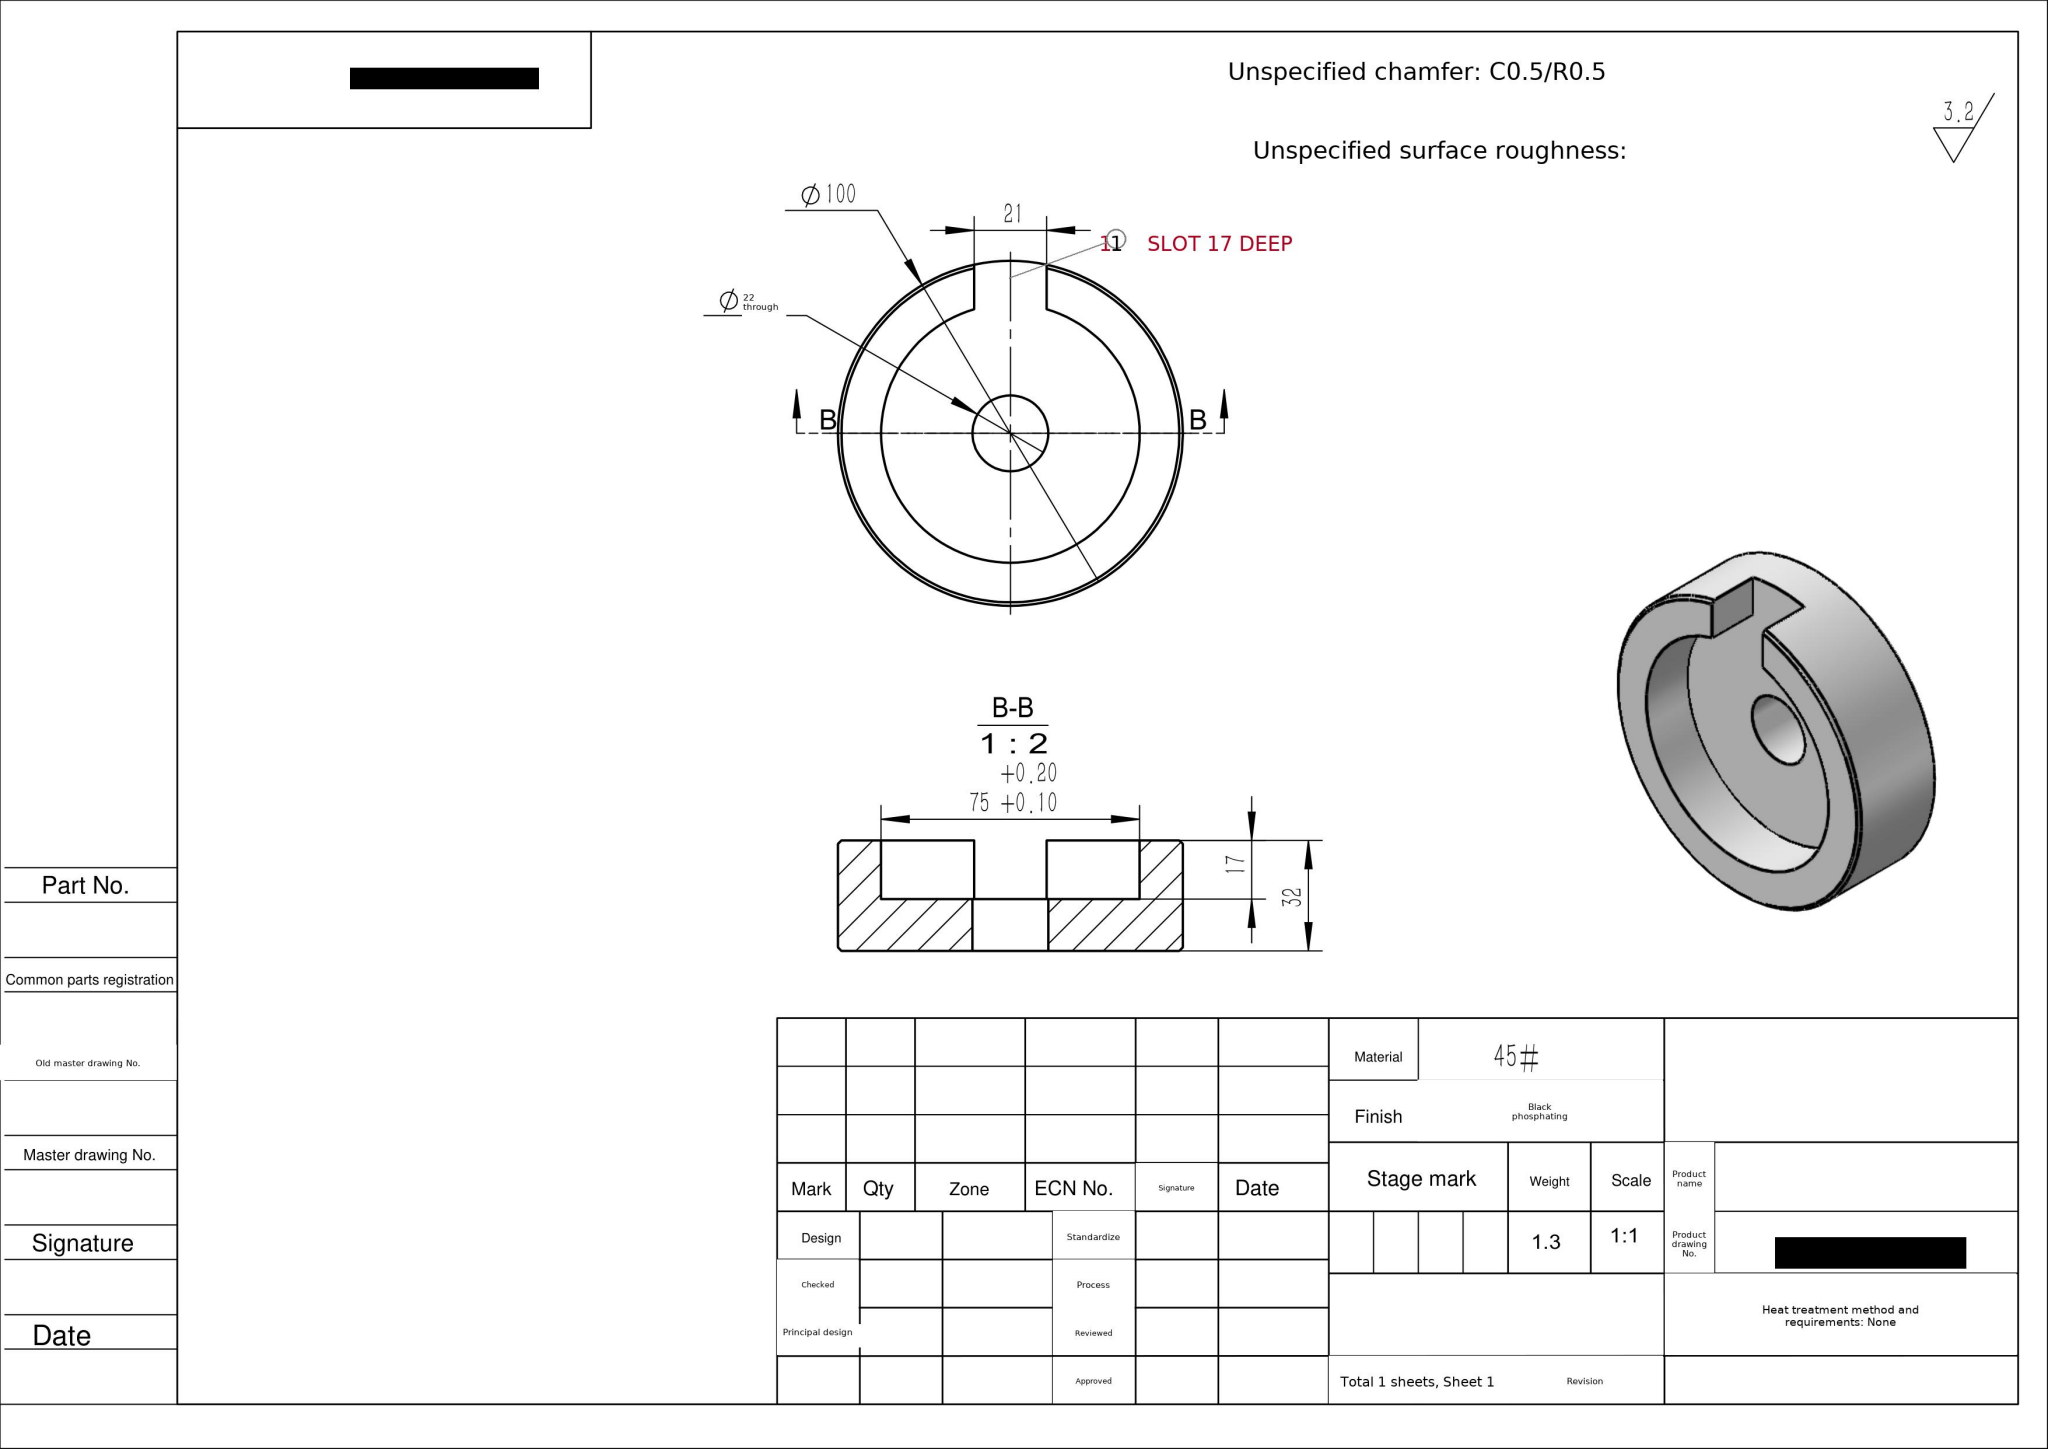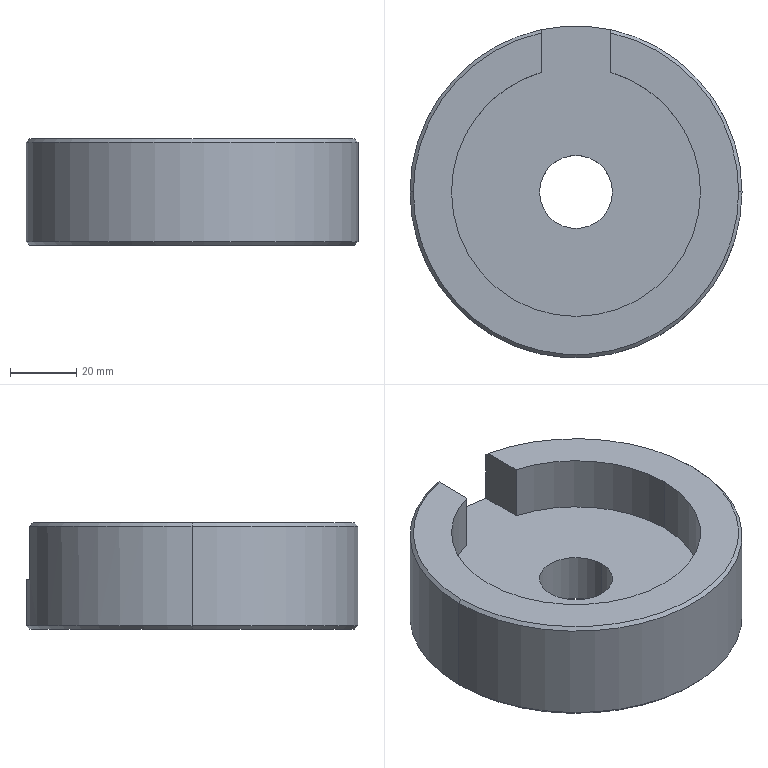Part | SolidWorks | mm | material 45# | 1 solid | 17 faces | box 100 x 100 x 32 mm | volume 165713 mm3 | cylinder 7 | cone 5 | plane 5 | commonest cylinder face diameters 75 x3 22 x2 100 x2
build123d program:
from build123d import *

# Parameters (mm, degrees)
SKETCH1_R             = 50
BOSS_EXTRUDE1_DEPTH   = 15
M20_CLEARANCE_HOLE1_D = 22
SKETCH4_R             = 50
SKETCH4_R_2           = 37.5
BOSS_EXTRUDE2_DEPTH   = 17
CHAMFER1_SIZE         = 1
SKETCH5_W             = 21
SKETCH5_H             = 65.178
CUT_EXTRUDE1_DEPTH    = 17


with BuildPart() as part:
    # Sketch1 → Boss-Extrude1 (new body)
    with BuildSketch(Plane.XY):
        Circle(SKETCH1_R)
    extrude(amount=BOSS_EXTRUDE1_DEPTH)

    # M20 Clearance Hole1 (through all)
    with Locations(Plane.XY.offset(15)):
        with Locations((0, 0)):
            Hole(M20_CLEARANCE_HOLE1_D / 2)

    # Sketch4 → Boss-Extrude2 (add)
    with BuildSketch(Plane.XY.offset(15)):
        Circle(SKETCH4_R)
        Circle(SKETCH4_R_2, mode=Mode.SUBTRACT)
    extrude(amount=BOSS_EXTRUDE2_DEPTH)

    # Chamfer1
    chamfer1_edges = [part.edges().sort_by_distance(p)[0] for p in [
        (-50, 0, 32),
        (-50, 0, 0),
    ]]
    chamfer(chamfer1_edges, length=CHAMFER1_SIZE)

    # Sketch5 → Cut-Extrude1 (cut)
    with BuildSketch(Plane.XY.offset(32)):
        with Locations((0, 32.589)):
            Rectangle(SKETCH5_W, SKETCH5_H)
    extrude(amount=-CUT_EXTRUDE1_DEPTH, mode=Mode.SUBTRACT)


solid = part.part
STEP:
#1=CARTESIAN_POINT('',(49.,0.,32.));
#2=VERTEX_POINT('',#1);
#3=CARTESIAN_POINT('',(10.5,47.862,32.));
#4=VERTEX_POINT('',#3);
#5=CARTESIAN_POINT('',(0.,0.,32.));
#6=DIRECTION('',(0.,0.,1.));
#7=DIRECTION('',(1.,0.,0.));
#8=AXIS2_PLACEMENT_3D('',#5,#6,#7);
#9=CIRCLE('',#8,49.);
#10=EDGE_CURVE('',#2,#4,#9,.T.);
#11=ORIENTED_EDGE('',*,*,#10,.F.);
#12=CARTESIAN_POINT('',(50.,0.,31.));
#13=VERTEX_POINT('',#12);
#14=CARTESIAN_POINT('',(49.,0.,32.));
#15=DIRECTION('',(0.7071,0.,-0.7071));
#16=VECTOR('',#15,1000.);
#17=LINE('',#14,#16);
#18=EDGE_CURVE('',#2,#13,#17,.T.);
#19=ORIENTED_EDGE('',*,*,#18,.T.);
#20=CARTESIAN_POINT('',(10.5,48.885,31.));
#21=VERTEX_POINT('',#20);
#22=CARTESIAN_POINT('',(0.,0.,31.));
#23=DIRECTION('',(0.,0.,-1.));
#24=DIRECTION('',(1.,0.,0.));
#25=AXIS2_PLACEMENT_3D('',#22,#23,#24);
#26=CIRCLE('',#25,50.);
#27=EDGE_CURVE('',#21,#13,#26,.T.);
#28=ORIENTED_EDGE('',*,*,#27,.F.);
#29=CARTESIAN_POINT('',(10.5,47.862,32.));
#30=CARTESIAN_POINT('',(10.5,48.203,31.667));
#31=CARTESIAN_POINT('',(10.5,48.544,31.333));
#32=CARTESIAN_POINT('',(10.5,48.885,31.));
#33=B_SPLINE_CURVE_WITH_KNOTS('',3,(#29,#30,#31,#32),.UNSPECIFIED.,.F.,.F.,(4,4),(0.04568,0.04711),.UNSPECIFIED.);
#34=EDGE_CURVE('',#4,#21,#33,.T.);
#35=ORIENTED_EDGE('',*,*,#34,.F.);
#36=EDGE_LOOP('',(#11,#19,#28,#35));
#37=FACE_OUTER_BOUND('',#36,.T.);
#38=CARTESIAN_POINT('',(0.,0.,32.));
#39=DIRECTION('',(0.,0.,-1.));
#40=DIRECTION('',(-1.,0.,0.));
#41=AXIS2_PLACEMENT_3D('',#38,#39,#40);
#42=CONICAL_SURFACE('',#41,49.,0.7854);
#43=ADVANCED_FACE('',(#37),#42,.T.);
#44=ORIENTED_EDGE('',*,*,#18,.F.);
#45=CARTESIAN_POINT('',(-49.,0.,32.));
#46=VERTEX_POINT('',#45);
#47=CARTESIAN_POINT('',(0.,0.,32.));
#48=DIRECTION('',(0.,0.,1.));
#49=DIRECTION('',(1.,0.,0.));
#50=AXIS2_PLACEMENT_3D('',#47,#48,#49);
#51=CIRCLE('',#50,49.);
#52=EDGE_CURVE('',#46,#2,#51,.T.);
#53=ORIENTED_EDGE('',*,*,#52,.F.);
#54=CARTESIAN_POINT('',(-50.,0.,31.));
#55=VERTEX_POINT('',#54);
#56=CARTESIAN_POINT('',(-49.,0.,32.));
#57=DIRECTION('',(-0.7071,0.,-0.7071));
#58=VECTOR('',#57,1000.);
#59=LINE('',#56,#58);
#60=EDGE_CURVE('',#46,#55,#59,.T.);
#61=ORIENTED_EDGE('',*,*,#60,.T.);
#62=CARTESIAN_POINT('',(0.,0.,31.));
#63=DIRECTION('',(0.,0.,-1.));
#64=DIRECTION('',(1.,0.,0.));
#65=AXIS2_PLACEMENT_3D('',#62,#63,#64);
#66=CIRCLE('',#65,50.);
#67=EDGE_CURVE('',#13,#55,#66,.T.);
#68=ORIENTED_EDGE('',*,*,#67,.F.);
#69=EDGE_LOOP('',(#44,#53,#61,#68));
#70=FACE_OUTER_BOUND('',#69,.T.);
#71=CARTESIAN_POINT('',(0.,0.,32.));
#72=DIRECTION('',(0.,0.,-1.));
#73=DIRECTION('',(-1.,0.,0.));
#74=AXIS2_PLACEMENT_3D('',#71,#72,#73);
#75=CONICAL_SURFACE('',#74,49.,0.7854);
#76=ADVANCED_FACE('',(#70),#75,.T.);
#77=CARTESIAN_POINT('',(-49.,0.,0.));
#78=VERTEX_POINT('',#77);
#79=CARTESIAN_POINT('',(49.,0.,0.));
#80=VERTEX_POINT('',#79);
#81=CARTESIAN_POINT('',(0.,0.,0.));
#82=DIRECTION('',(0.,0.,-1.));
#83=DIRECTION('',(1.,0.,0.));
#84=AXIS2_PLACEMENT_3D('',#81,#82,#83);
#85=CIRCLE('',#84,49.);
#86=EDGE_CURVE('',#78,#80,#85,.T.);
#87=ORIENTED_EDGE('',*,*,#86,.F.);
#88=CARTESIAN_POINT('',(-50.,0.,1.));
#89=VERTEX_POINT('',#88);
#90=CARTESIAN_POINT('',(-50.,0.,1.));
#91=DIRECTION('',(-0.7071,0.,0.7071));
#92=VECTOR('',#91,1000.);
#93=LINE('',#90,#92);
#94=EDGE_CURVE('',#78,#89,#93,.T.);
#95=ORIENTED_EDGE('',*,*,#94,.T.);
#96=CARTESIAN_POINT('',(50.,0.,1.));
#97=VERTEX_POINT('',#96);
#98=CARTESIAN_POINT('',(0.,0.,1.));
#99=DIRECTION('',(0.,0.,1.));
#100=DIRECTION('',(1.,0.,0.));
#101=AXIS2_PLACEMENT_3D('',#98,#99,#100);
#102=CIRCLE('',#101,50.);
#103=EDGE_CURVE('',#97,#89,#102,.T.);
#104=ORIENTED_EDGE('',*,*,#103,.F.);
#105=CARTESIAN_POINT('',(50.,0.,1.));
#106=DIRECTION('',(0.7071,0.,0.7071));
#107=VECTOR('',#106,1000.);
#108=LINE('',#105,#107);
#109=EDGE_CURVE('',#80,#97,#108,.T.);
#110=ORIENTED_EDGE('',*,*,#109,.F.);
#111=EDGE_LOOP('',(#87,#95,#104,#110));
#112=FACE_OUTER_BOUND('',#111,.T.);
#113=CARTESIAN_POINT('',(0.,0.,1.));
#114=DIRECTION('',(0.,0.,1.));
#115=DIRECTION('',(1.,0.,0.));
#116=AXIS2_PLACEMENT_3D('',#113,#114,#115);
#117=CONICAL_SURFACE('',#116,50.,0.7854);
#118=ADVANCED_FACE('',(#112),#117,.T.);
#119=CARTESIAN_POINT('',(-37.5,0.,32.));
#120=VERTEX_POINT('',#119);
#121=CARTESIAN_POINT('',(37.5,0.,32.));
#122=VERTEX_POINT('',#121);
#123=CARTESIAN_POINT('',(0.,0.,32.));
#124=DIRECTION('',(0.,0.,1.));
#125=DIRECTION('',(1.,0.,0.));
#126=AXIS2_PLACEMENT_3D('',#123,#124,#125);
#127=CIRCLE('',#126,37.5);
#128=EDGE_CURVE('',#120,#122,#127,.T.);
#129=ORIENTED_EDGE('',*,*,#128,.T.);
#130=CARTESIAN_POINT('',(37.5,0.,15.));
#131=VERTEX_POINT('',#130);
#132=CARTESIAN_POINT('',(37.5,0.,32.));
#133=DIRECTION('',(0.,0.,-1.));
#134=VECTOR('',#133,1000.);
#135=LINE('',#132,#134);
#136=EDGE_CURVE('',#122,#131,#135,.T.);
#137=ORIENTED_EDGE('',*,*,#136,.T.);
#138=CARTESIAN_POINT('',(-37.5,0.,15.));
#139=VERTEX_POINT('',#138);
#140=CARTESIAN_POINT('',(0.,0.,15.));
#141=DIRECTION('',(0.,0.,-1.));
#142=DIRECTION('',(1.,0.,0.));
#143=AXIS2_PLACEMENT_3D('',#140,#141,#142);
#144=CIRCLE('',#143,37.5);
#145=EDGE_CURVE('',#131,#139,#144,.T.);
#146=ORIENTED_EDGE('',*,*,#145,.T.);
#147=CARTESIAN_POINT('',(-37.5,0.,32.));
#148=DIRECTION('',(0.,0.,-1.));
#149=VECTOR('',#148,1000.);
#150=LINE('',#147,#149);
#151=EDGE_CURVE('',#120,#139,#150,.T.);
#152=ORIENTED_EDGE('',*,*,#151,.F.);
#153=EDGE_LOOP('',(#129,#137,#146,#152));
#154=FACE_OUTER_BOUND('',#153,.T.);
#155=CARTESIAN_POINT('',(0.,0.,32.));
#156=DIRECTION('',(0.,0.,-1.));
#157=DIRECTION('',(-1.,0.,0.));
#158=AXIS2_PLACEMENT_3D('',#155,#156,#157);
#159=CYLINDRICAL_SURFACE('',#158,37.5);
#160=ADVANCED_FACE('',(#154),#159,.F.);
#161=CARTESIAN_POINT('',(-10.5,36.,32.));
#162=VERTEX_POINT('',#161);
#163=CARTESIAN_POINT('',(0.,0.,32.));
#164=DIRECTION('',(0.,0.,1.));
#165=DIRECTION('',(1.,0.,0.));
#166=AXIS2_PLACEMENT_3D('',#163,#164,#165);
#167=CIRCLE('',#166,37.5);
#168=EDGE_CURVE('',#162,#120,#167,.T.);
#169=ORIENTED_EDGE('',*,*,#168,.T.);
#170=ORIENTED_EDGE('',*,*,#151,.T.);
#171=CARTESIAN_POINT('',(-10.5,36.,15.));
#172=VERTEX_POINT('',#171);
#173=CARTESIAN_POINT('',(0.,0.,15.));
#174=DIRECTION('',(0.,0.,-1.));
#175=DIRECTION('',(1.,0.,0.));
#176=AXIS2_PLACEMENT_3D('',#173,#174,#175);
#177=CIRCLE('',#176,37.5);
#178=EDGE_CURVE('',#139,#172,#177,.T.);
#179=ORIENTED_EDGE('',*,*,#178,.T.);
#180=CARTESIAN_POINT('',(-10.5,36.,32.));
#181=DIRECTION('',(0.,0.,-1.));
#182=VECTOR('',#181,1000.);
#183=LINE('',#180,#182);
#184=EDGE_CURVE('',#162,#172,#183,.T.);
#185=ORIENTED_EDGE('',*,*,#184,.F.);
#186=EDGE_LOOP('',(#169,#170,#179,#185));
#187=FACE_OUTER_BOUND('',#186,.T.);
#188=CARTESIAN_POINT('',(0.,0.,32.));
#189=DIRECTION('',(0.,0.,-1.));
#190=DIRECTION('',(-1.,0.,0.));
#191=AXIS2_PLACEMENT_3D('',#188,#189,#190);
#192=CYLINDRICAL_SURFACE('',#191,37.5);
#193=ADVANCED_FACE('',(#187),#192,.F.);
#194=CARTESIAN_POINT('',(-11.,0.,0.));
#195=VERTEX_POINT('',#194);
#196=CARTESIAN_POINT('',(11.,0.,0.));
#197=VERTEX_POINT('',#196);
#198=CARTESIAN_POINT('',(0.,0.,0.));
#199=DIRECTION('',(0.,0.,1.));
#200=DIRECTION('',(1.,0.,0.));
#201=AXIS2_PLACEMENT_3D('',#198,#199,#200);
#202=CIRCLE('',#201,11.);
#203=EDGE_CURVE('',#195,#197,#202,.T.);
#204=ORIENTED_EDGE('',*,*,#203,.F.);
#205=CARTESIAN_POINT('',(-11.,0.,15.));
#206=VERTEX_POINT('',#205);
#207=CARTESIAN_POINT('',(-11.,0.,15.));
#208=DIRECTION('',(0.,0.,1.));
#209=VECTOR('',#208,1000.);
#210=LINE('',#207,#209);
#211=EDGE_CURVE('',#195,#206,#210,.T.);
#212=ORIENTED_EDGE('',*,*,#211,.T.);
#213=CARTESIAN_POINT('',(11.,0.,15.));
#214=VERTEX_POINT('',#213);
#215=CARTESIAN_POINT('',(0.,0.,15.));
#216=DIRECTION('',(0.,0.,1.));
#217=DIRECTION('',(1.,0.,0.));
#218=AXIS2_PLACEMENT_3D('',#215,#216,#217);
#219=CIRCLE('',#218,11.);
#220=EDGE_CURVE('',#206,#214,#219,.T.);
#221=ORIENTED_EDGE('',*,*,#220,.T.);
#222=CARTESIAN_POINT('',(11.,0.,15.));
#223=DIRECTION('',(0.,0.,1.));
#224=VECTOR('',#223,1000.);
#225=LINE('',#222,#224);
#226=EDGE_CURVE('',#197,#214,#225,.T.);
#227=ORIENTED_EDGE('',*,*,#226,.F.);
#228=EDGE_LOOP('',(#204,#212,#221,#227));
#229=FACE_OUTER_BOUND('',#228,.T.);
#230=CARTESIAN_POINT('',(0.,0.,15.));
#231=DIRECTION('',(0.,0.,1.));
#232=DIRECTION('',(1.,0.,0.));
#233=AXIS2_PLACEMENT_3D('',#230,#231,#232);
#234=CYLINDRICAL_SURFACE('',#233,11.);
#235=ADVANCED_FACE('',(#229),#234,.F.);
#236=ORIENTED_EDGE('',*,*,#27,.T.);
#237=CARTESIAN_POINT('',(50.,0.,15.));
#238=DIRECTION('',(0.,0.,-1.));
#239=VECTOR('',#238,1000.);
#240=LINE('',#237,#239);
#241=EDGE_CURVE('',#13,#97,#240,.T.);
#242=ORIENTED_EDGE('',*,*,#241,.T.);
#243=ORIENTED_EDGE('',*,*,#103,.T.);
#244=CARTESIAN_POINT('',(-50.,0.,15.));
#245=DIRECTION('',(0.,0.,-1.));
#246=VECTOR('',#245,1000.);
#247=LINE('',#244,#246);
#248=EDGE_CURVE('',#55,#89,#247,.T.);
#249=ORIENTED_EDGE('',*,*,#248,.F.);
#250=CARTESIAN_POINT('',(-10.5,48.885,31.));
#251=VERTEX_POINT('',#250);
#252=CARTESIAN_POINT('',(0.,0.,31.));
#253=DIRECTION('',(0.,0.,-1.));
#254=DIRECTION('',(1.,0.,0.));
#255=AXIS2_PLACEMENT_3D('',#252,#253,#254);
#256=CIRCLE('',#255,50.);
#257=EDGE_CURVE('',#55,#251,#256,.T.);
#258=ORIENTED_EDGE('',*,*,#257,.T.);
#259=CARTESIAN_POINT('',(-10.5,48.885,15.));
#260=VERTEX_POINT('',#259);
#261=CARTESIAN_POINT('',(-10.5,48.885,15.));
#262=DIRECTION('',(0.,0.,-1.));
#263=VECTOR('',#262,1000.);
#264=LINE('',#261,#263);
#265=EDGE_CURVE('',#251,#260,#264,.T.);
#266=ORIENTED_EDGE('',*,*,#265,.T.);
#267=CARTESIAN_POINT('',(10.5,48.885,15.));
#268=VERTEX_POINT('',#267);
#269=CARTESIAN_POINT('',(0.,0.,15.));
#270=DIRECTION('',(0.,0.,1.));
#271=DIRECTION('',(1.,0.,0.));
#272=AXIS2_PLACEMENT_3D('',#269,#270,#271);
#273=CIRCLE('',#272,50.);
#274=EDGE_CURVE('',#268,#260,#273,.T.);
#275=ORIENTED_EDGE('',*,*,#274,.F.);
#276=CARTESIAN_POINT('',(10.5,48.885,15.));
#277=DIRECTION('',(0.,0.,1.));
#278=VECTOR('',#277,1000.);
#279=LINE('',#276,#278);
#280=EDGE_CURVE('',#268,#21,#279,.T.);
#281=ORIENTED_EDGE('',*,*,#280,.T.);
#282=EDGE_LOOP('',(#236,#242,#243,#249,#258,#266,#275,#281));
#283=FACE_OUTER_BOUND('',#282,.T.);
#284=CARTESIAN_POINT('',(0.,0.,15.));
#285=DIRECTION('',(0.,0.,-1.));
#286=DIRECTION('',(-1.,0.,0.));
#287=AXIS2_PLACEMENT_3D('',#284,#285,#286);
#288=CYLINDRICAL_SURFACE('',#287,50.);
#289=ADVANCED_FACE('',(#283),#288,.T.);
#290=CARTESIAN_POINT('',(10.5,36.,15.));
#291=VERTEX_POINT('',#290);
#292=CARTESIAN_POINT('',(0.,0.,15.));
#293=DIRECTION('',(0.,0.,-1.));
#294=DIRECTION('',(1.,0.,0.));
#295=AXIS2_PLACEMENT_3D('',#292,#293,#294);
#296=CIRCLE('',#295,37.5);
#297=EDGE_CURVE('',#291,#131,#296,.T.);
#298=ORIENTED_EDGE('',*,*,#297,.F.);
#299=CARTESIAN_POINT('',(10.5,-0.,15.));
#300=DIRECTION('',(-0.,-1.,0.));
#301=VECTOR('',#300,1000.);
#302=LINE('',#299,#301);
#303=EDGE_CURVE('',#268,#291,#302,.T.);
#304=ORIENTED_EDGE('',*,*,#303,.F.);
#305=ORIENTED_EDGE('',*,*,#274,.T.);
#306=CARTESIAN_POINT('',(-10.5,-0.,15.));
#307=DIRECTION('',(-0.,1.,0.));
#308=VECTOR('',#307,1000.);
#309=LINE('',#306,#308);
#310=EDGE_CURVE('',#172,#260,#309,.T.);
#311=ORIENTED_EDGE('',*,*,#310,.F.);
#312=ORIENTED_EDGE('',*,*,#178,.F.);
#313=ORIENTED_EDGE('',*,*,#145,.F.);
#314=EDGE_LOOP('',(#298,#304,#305,#311,#312,#313));
#315=FACE_OUTER_BOUND('',#314,.T.);
#316=CARTESIAN_POINT('',(0.,0.,15.));
#317=DIRECTION('',(0.,0.,1.));
#318=DIRECTION('',(1.,0.,0.));
#319=AXIS2_PLACEMENT_3D('',#316,#317,#318);
#320=CIRCLE('',#319,11.);
#321=EDGE_CURVE('',#214,#206,#320,.T.);
#322=ORIENTED_EDGE('',*,*,#321,.F.);
#323=ORIENTED_EDGE('',*,*,#220,.F.);
#324=EDGE_LOOP('',(#322,#323));
#325=FACE_BOUND('',#324,.T.);
#326=CARTESIAN_POINT('',(0.,0.,15.));
#327=DIRECTION('',(0.,0.,1.));
#328=DIRECTION('',(1.,0.,0.));
#329=AXIS2_PLACEMENT_3D('',#326,#327,#328);
#330=PLANE('',#329);
#331=ADVANCED_FACE('',(#315,#325),#330,.T.);
#332=ORIENTED_EDGE('',*,*,#241,.F.);
#333=ORIENTED_EDGE('',*,*,#67,.T.);
#334=ORIENTED_EDGE('',*,*,#248,.T.);
#335=CARTESIAN_POINT('',(0.,0.,1.));
#336=DIRECTION('',(0.,0.,1.));
#337=DIRECTION('',(1.,0.,0.));
#338=AXIS2_PLACEMENT_3D('',#335,#336,#337);
#339=CIRCLE('',#338,50.);
#340=EDGE_CURVE('',#89,#97,#339,.T.);
#341=ORIENTED_EDGE('',*,*,#340,.T.);
#342=EDGE_LOOP('',(#332,#333,#334,#341));
#343=FACE_OUTER_BOUND('',#342,.T.);
#344=CARTESIAN_POINT('',(0.,0.,15.));
#345=DIRECTION('',(0.,0.,-1.));
#346=DIRECTION('',(-1.,0.,0.));
#347=AXIS2_PLACEMENT_3D('',#344,#345,#346);
#348=CYLINDRICAL_SURFACE('',#347,50.);
#349=ADVANCED_FACE('',(#343),#348,.T.);
#350=CARTESIAN_POINT('',(0.,0.,0.));
#351=DIRECTION('',(0.,0.,-1.));
#352=DIRECTION('',(1.,0.,0.));
#353=AXIS2_PLACEMENT_3D('',#350,#351,#352);
#354=CIRCLE('',#353,49.);
#355=EDGE_CURVE('',#80,#78,#354,.T.);
#356=ORIENTED_EDGE('',*,*,#355,.T.);
#357=ORIENTED_EDGE('',*,*,#86,.T.);
#358=EDGE_LOOP('',(#356,#357));
#359=FACE_OUTER_BOUND('',#358,.T.);
#360=CARTESIAN_POINT('',(0.,0.,0.));
#361=DIRECTION('',(0.,0.,1.));
#362=DIRECTION('',(1.,0.,0.));
#363=AXIS2_PLACEMENT_3D('',#360,#361,#362);
#364=CIRCLE('',#363,11.);
#365=EDGE_CURVE('',#197,#195,#364,.T.);
#366=ORIENTED_EDGE('',*,*,#365,.T.);
#367=ORIENTED_EDGE('',*,*,#203,.T.);
#368=EDGE_LOOP('',(#366,#367));
#369=FACE_BOUND('',#368,.T.);
#370=CARTESIAN_POINT('',(0.,0.,0.));
#371=DIRECTION('',(0.,0.,1.));
#372=DIRECTION('',(1.,0.,0.));
#373=AXIS2_PLACEMENT_3D('',#370,#371,#372);
#374=PLANE('',#373);
#375=ADVANCED_FACE('',(#359,#369),#374,.F.);
#376=ORIENTED_EDGE('',*,*,#211,.F.);
#377=ORIENTED_EDGE('',*,*,#365,.F.);
#378=ORIENTED_EDGE('',*,*,#226,.T.);
#379=ORIENTED_EDGE('',*,*,#321,.T.);
#380=EDGE_LOOP('',(#376,#377,#378,#379));
#381=FACE_OUTER_BOUND('',#380,.T.);
#382=CARTESIAN_POINT('',(0.,0.,15.));
#383=DIRECTION('',(0.,0.,1.));
#384=DIRECTION('',(1.,0.,0.));
#385=AXIS2_PLACEMENT_3D('',#382,#383,#384);
#386=CYLINDRICAL_SURFACE('',#385,11.);
#387=ADVANCED_FACE('',(#381),#386,.F.);
#388=CARTESIAN_POINT('',(10.5,36.,32.));
#389=VERTEX_POINT('',#388);
#390=CARTESIAN_POINT('',(10.5,-0.,32.));
#391=DIRECTION('',(0.,1.,0.));
#392=VECTOR('',#391,1000.);
#393=LINE('',#390,#392);
#394=EDGE_CURVE('',#389,#4,#393,.T.);
#395=ORIENTED_EDGE('',*,*,#394,.F.);
#396=CARTESIAN_POINT('',(0.,0.,32.));
#397=DIRECTION('',(0.,0.,1.));
#398=DIRECTION('',(1.,0.,0.));
#399=AXIS2_PLACEMENT_3D('',#396,#397,#398);
#400=CIRCLE('',#399,37.5);
#401=EDGE_CURVE('',#122,#389,#400,.T.);
#402=ORIENTED_EDGE('',*,*,#401,.F.);
#403=ORIENTED_EDGE('',*,*,#128,.F.);
#404=ORIENTED_EDGE('',*,*,#168,.F.);
#405=CARTESIAN_POINT('',(-10.5,47.862,32.));
#406=VERTEX_POINT('',#405);
#407=CARTESIAN_POINT('',(-10.5,-0.,32.));
#408=DIRECTION('',(0.,-1.,0.));
#409=VECTOR('',#408,1000.);
#410=LINE('',#407,#409);
#411=EDGE_CURVE('',#406,#162,#410,.T.);
#412=ORIENTED_EDGE('',*,*,#411,.F.);
#413=CARTESIAN_POINT('',(0.,0.,32.));
#414=DIRECTION('',(0.,0.,1.));
#415=DIRECTION('',(1.,0.,0.));
#416=AXIS2_PLACEMENT_3D('',#413,#414,#415);
#417=CIRCLE('',#416,49.);
#418=EDGE_CURVE('',#406,#46,#417,.T.);
#419=ORIENTED_EDGE('',*,*,#418,.T.);
#420=ORIENTED_EDGE('',*,*,#52,.T.);
#421=ORIENTED_EDGE('',*,*,#10,.T.);
#422=EDGE_LOOP('',(#395,#402,#403,#404,#412,#419,#420,#421));
#423=FACE_OUTER_BOUND('',#422,.T.);
#424=CARTESIAN_POINT('',(0.,0.,32.));
#425=DIRECTION('',(0.,0.,1.));
#426=DIRECTION('',(1.,0.,0.));
#427=AXIS2_PLACEMENT_3D('',#424,#425,#426);
#428=PLANE('',#427);
#429=ADVANCED_FACE('',(#423),#428,.T.);
#430=ORIENTED_EDGE('',*,*,#136,.F.);
#431=ORIENTED_EDGE('',*,*,#401,.T.);
#432=CARTESIAN_POINT('',(10.5,36.,32.));
#433=DIRECTION('',(0.,0.,1.));
#434=VECTOR('',#433,1000.);
#435=LINE('',#432,#434);
#436=EDGE_CURVE('',#291,#389,#435,.T.);
#437=ORIENTED_EDGE('',*,*,#436,.F.);
#438=ORIENTED_EDGE('',*,*,#297,.T.);
#439=EDGE_LOOP('',(#430,#431,#437,#438));
#440=FACE_OUTER_BOUND('',#439,.T.);
#441=CARTESIAN_POINT('',(0.,0.,32.));
#442=DIRECTION('',(0.,0.,-1.));
#443=DIRECTION('',(-1.,0.,0.));
#444=AXIS2_PLACEMENT_3D('',#441,#442,#443);
#445=CYLINDRICAL_SURFACE('',#444,37.5);
#446=ADVANCED_FACE('',(#440),#445,.F.);
#447=ORIENTED_EDGE('',*,*,#94,.F.);
#448=ORIENTED_EDGE('',*,*,#355,.F.);
#449=ORIENTED_EDGE('',*,*,#109,.T.);
#450=ORIENTED_EDGE('',*,*,#340,.F.);
#451=EDGE_LOOP('',(#447,#448,#449,#450));
#452=FACE_OUTER_BOUND('',#451,.T.);
#453=CARTESIAN_POINT('',(0.,0.,1.));
#454=DIRECTION('',(0.,0.,1.));
#455=DIRECTION('',(1.,0.,0.));
#456=AXIS2_PLACEMENT_3D('',#453,#454,#455);
#457=CONICAL_SURFACE('',#456,50.,0.7854);
#458=ADVANCED_FACE('',(#452),#457,.T.);
#459=ORIENTED_EDGE('',*,*,#60,.F.);
#460=ORIENTED_EDGE('',*,*,#418,.F.);
#461=CARTESIAN_POINT('',(-10.5,48.885,31.));
#462=CARTESIAN_POINT('',(-10.5,48.544,31.333));
#463=CARTESIAN_POINT('',(-10.5,48.203,31.667));
#464=CARTESIAN_POINT('',(-10.5,47.862,32.));
#465=B_SPLINE_CURVE_WITH_KNOTS('',3,(#461,#462,#463,#464),.UNSPECIFIED.,.F.,.F.,(4,4),(0.05125,0.05268),.UNSPECIFIED.);
#466=EDGE_CURVE('',#251,#406,#465,.T.);
#467=ORIENTED_EDGE('',*,*,#466,.F.);
#468=ORIENTED_EDGE('',*,*,#257,.F.);
#469=EDGE_LOOP('',(#459,#460,#467,#468));
#470=FACE_OUTER_BOUND('',#469,.T.);
#471=CARTESIAN_POINT('',(0.,0.,32.));
#472=DIRECTION('',(0.,0.,-1.));
#473=DIRECTION('',(-1.,0.,0.));
#474=AXIS2_PLACEMENT_3D('',#471,#472,#473);
#475=CONICAL_SURFACE('',#474,49.,0.7854);
#476=ADVANCED_FACE('',(#470),#475,.T.);
#477=ORIENTED_EDGE('',*,*,#436,.T.);
#478=ORIENTED_EDGE('',*,*,#394,.T.);
#479=ORIENTED_EDGE('',*,*,#34,.T.);
#480=ORIENTED_EDGE('',*,*,#280,.F.);
#481=ORIENTED_EDGE('',*,*,#303,.T.);
#482=EDGE_LOOP('',(#477,#478,#479,#480,#481));
#483=FACE_OUTER_BOUND('',#482,.T.);
#484=CARTESIAN_POINT('',(10.5,-0.,-53.478));
#485=DIRECTION('',(1.,-0.,0.));
#486=DIRECTION('',(0.,1.,0.));
#487=AXIS2_PLACEMENT_3D('',#484,#485,#486);
#488=PLANE('',#487);
#489=ADVANCED_FACE('',(#483),#488,.F.);
#490=ORIENTED_EDGE('',*,*,#184,.T.);
#491=ORIENTED_EDGE('',*,*,#310,.T.);
#492=ORIENTED_EDGE('',*,*,#265,.F.);
#493=ORIENTED_EDGE('',*,*,#466,.T.);
#494=ORIENTED_EDGE('',*,*,#411,.T.);
#495=EDGE_LOOP('',(#490,#491,#492,#493,#494));
#496=FACE_OUTER_BOUND('',#495,.T.);
#497=CARTESIAN_POINT('',(-10.5,-0.,-53.478));
#498=DIRECTION('',(-1.,-0.,0.));
#499=DIRECTION('',(0.,-1.,0.));
#500=AXIS2_PLACEMENT_3D('',#497,#498,#499);
#501=PLANE('',#500);
#502=ADVANCED_FACE('',(#496),#501,.F.);
#503=CLOSED_SHELL('',(#43,#76,#118,#160,#193,#235,#289,#331,#349,#375,#387,#429,#446,#458,#476,#489,#502));
#504=MANIFOLD_SOLID_BREP('',#503);
#505=CARTESIAN_POINT('',(0.,0.,0.));
#506=DIRECTION('',(0.,0.,1.));
#507=DIRECTION('',(1.,0.,0.));
#508=AXIS2_PLACEMENT_3D('',#505,#506,#507);
#509=(LENGTH_UNIT()NAMED_UNIT(*)SI_UNIT(.MILLI.,.METRE.));
#510=UNCERTAINTY_MEASURE_WITH_UNIT(LENGTH_MEASURE(0.00001),#509,'','');
#511=(NAMED_UNIT(*)PLANE_ANGLE_UNIT()SI_UNIT($,.RADIAN.));
#512=(NAMED_UNIT(*)SI_UNIT($,.STERADIAN.)SOLID_ANGLE_UNIT());
#513=(GEOMETRIC_REPRESENTATION_CONTEXT(3)GLOBAL_UNCERTAINTY_ASSIGNED_CONTEXT((#510))GLOBAL_UNIT_ASSIGNED_CONTEXT((#509,#511,#512))REPRESENTATION_CONTEXT('',''));
#514=ADVANCED_BREP_SHAPE_REPRESENTATION('',(#504,#508),#513);